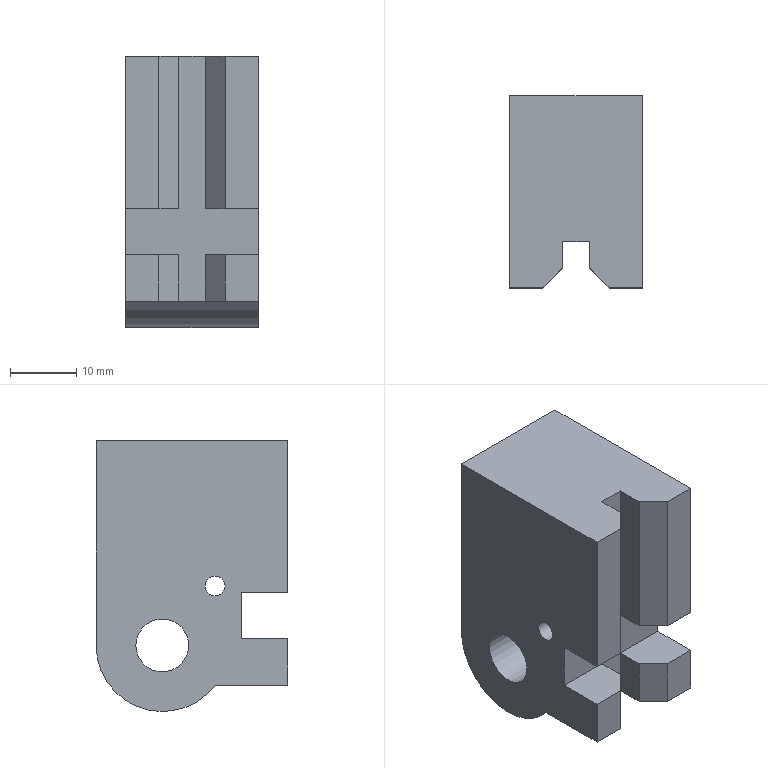Component | NX | CLAMP_BLOCK | 1 solid | 25 faces | volume 19041 mm3 | plane 22 | cylinder 3 | commonest cylinder face diameters 20 x1 3 x1 8 x1